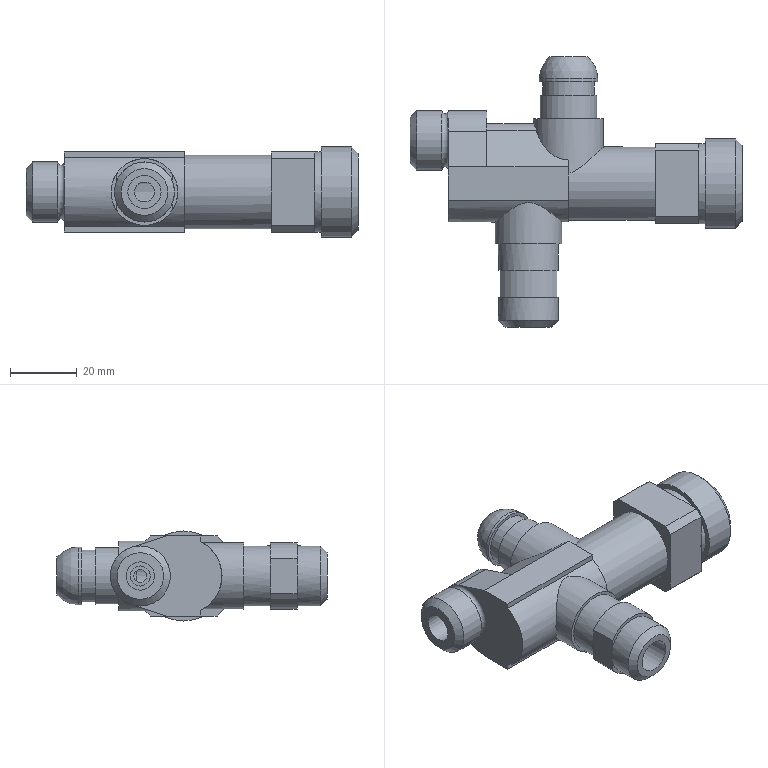Component | NX | FOUR_WAY_VALVE_BODY | 1 solid | 99 faces | volume 35096 mm3 | plane 59 | cylinder 35 | cone 3 | torus 1 | sphere 1 | commonest cylinder face diameters 18 x5 10 x5 20 x4 17 x2 16 x2 16.5 x2 6 x2 12 x2